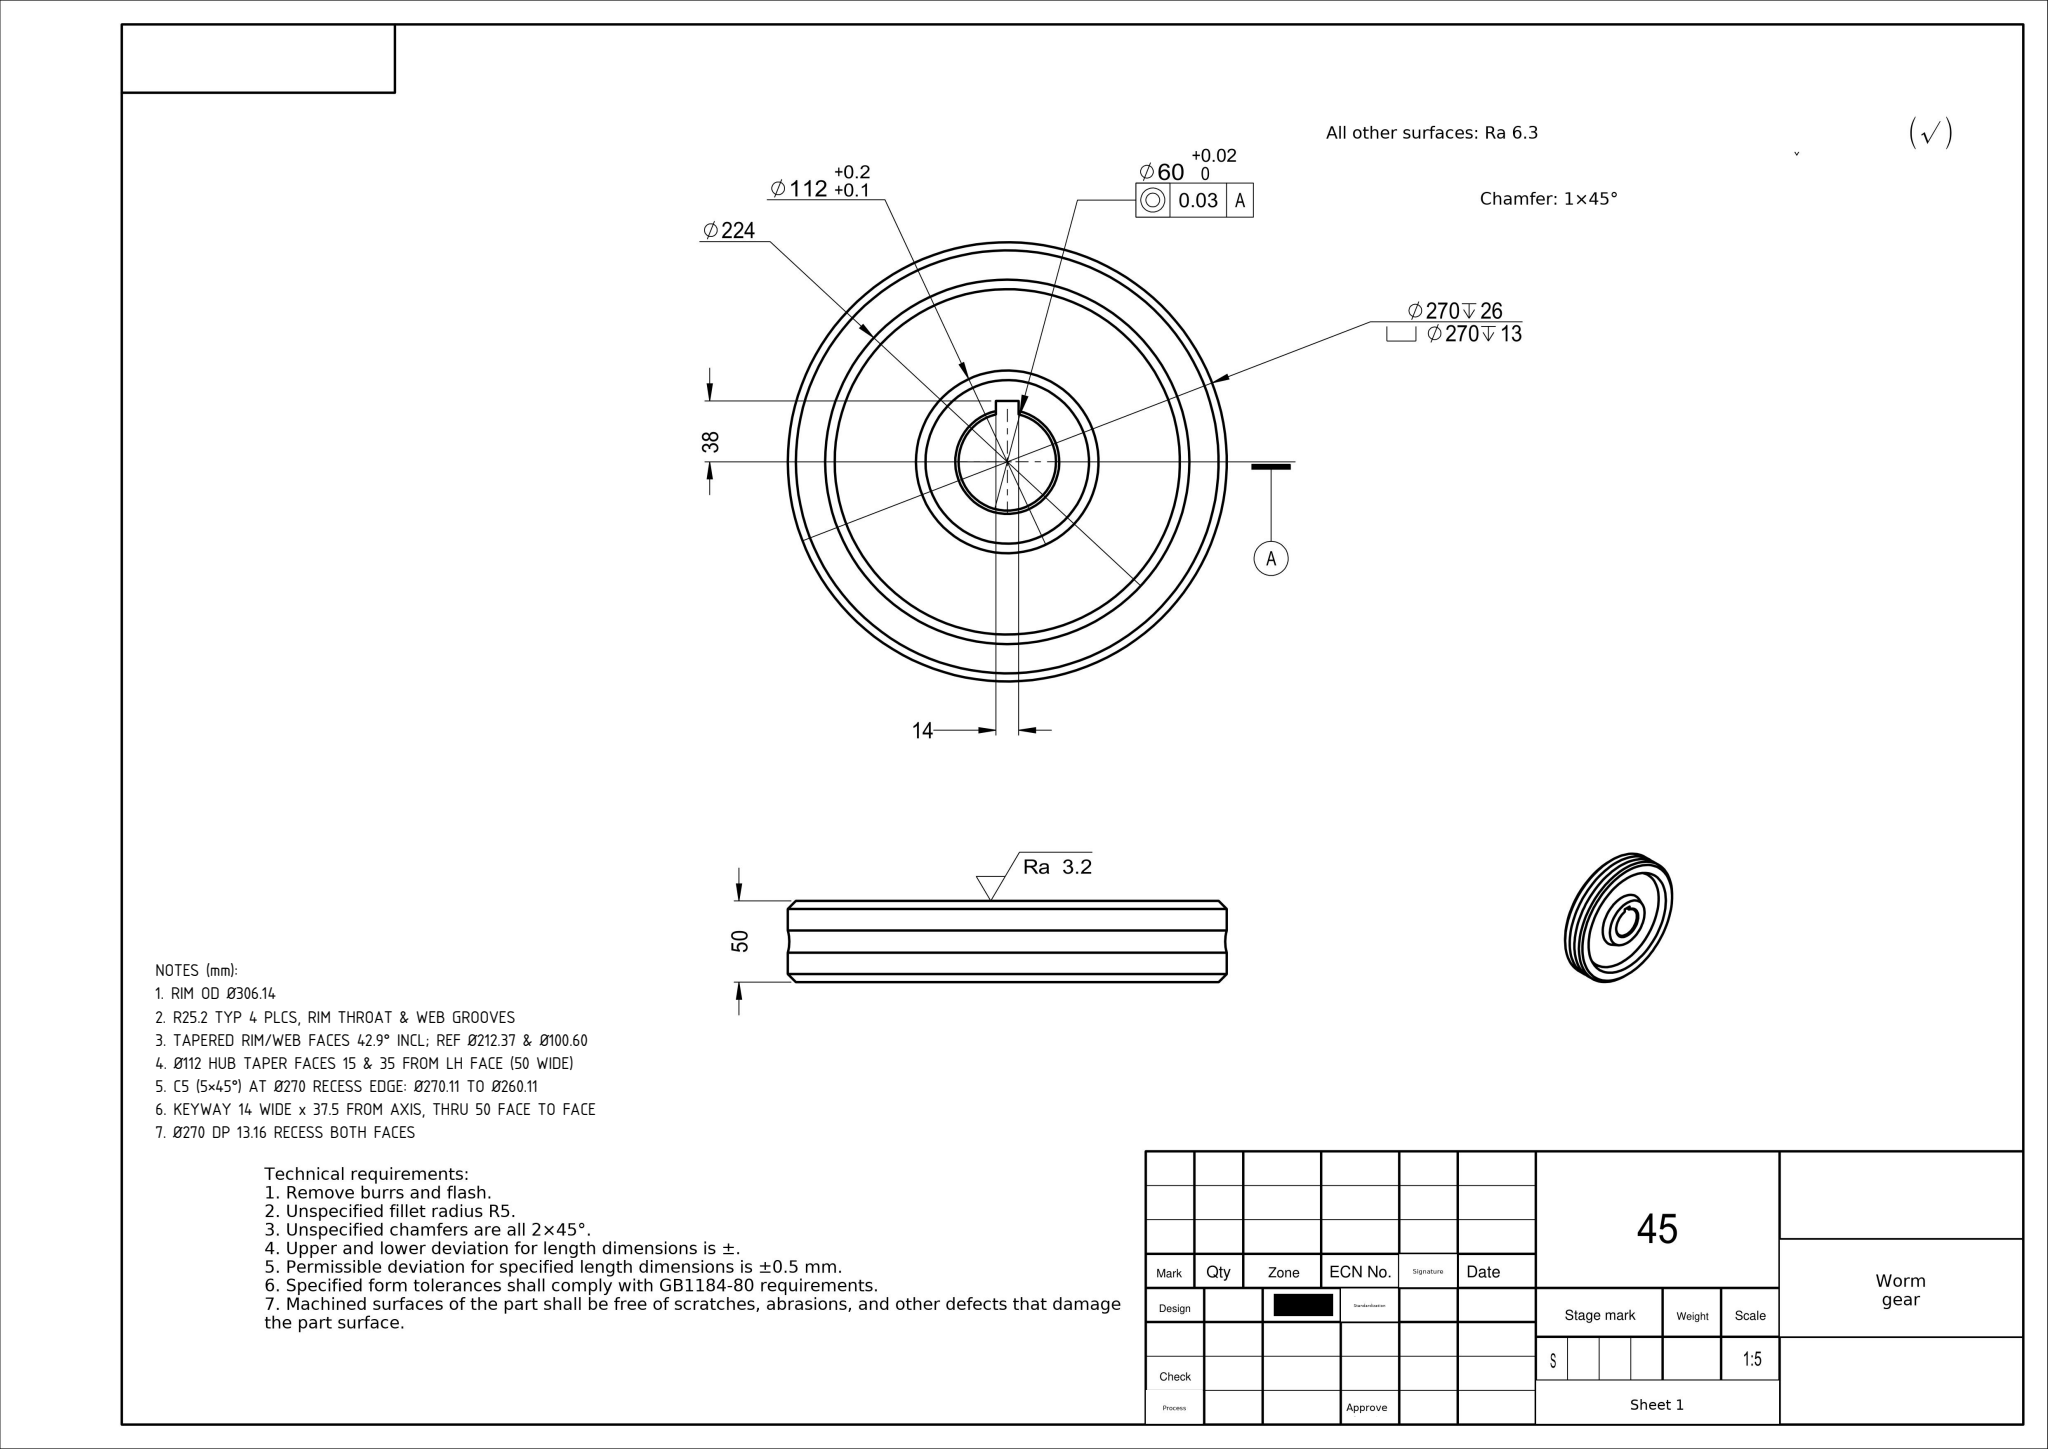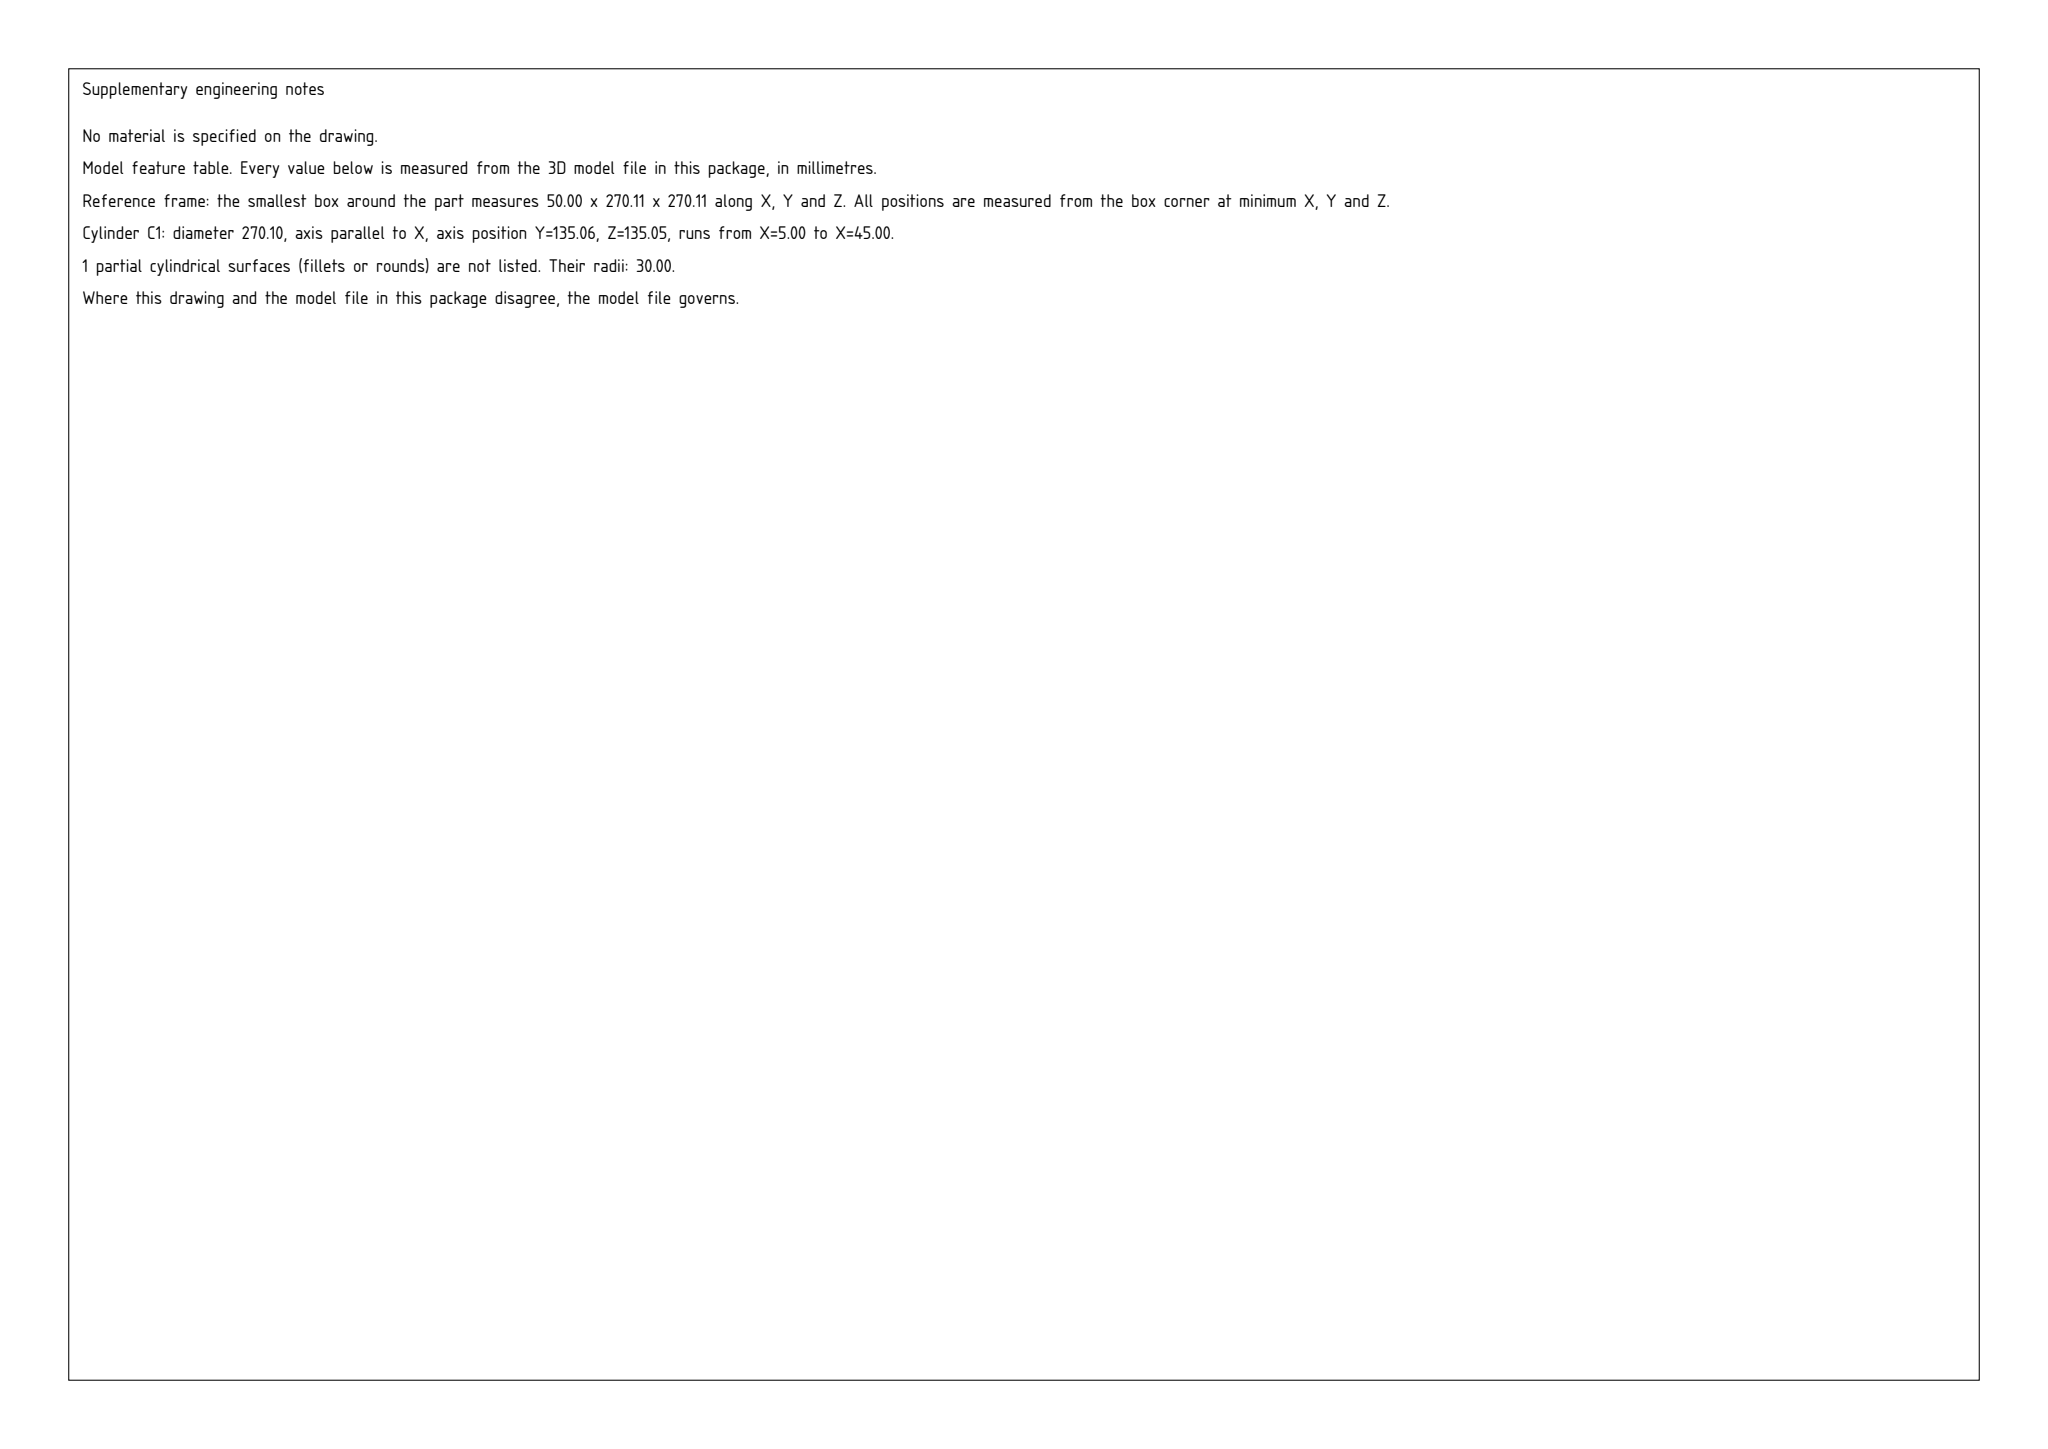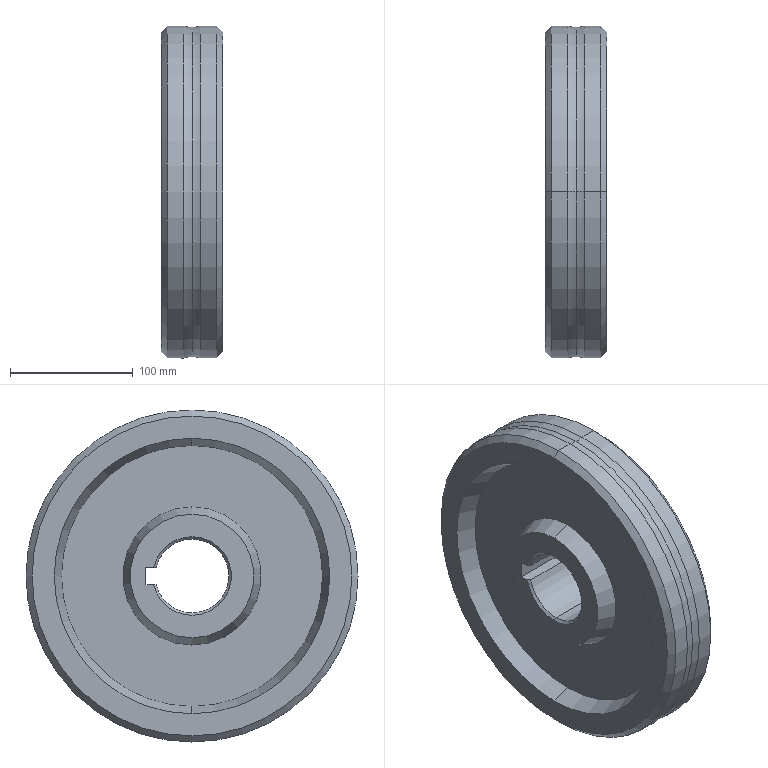Part | SolidWorks | mm | 1 solid | 38 faces | box 50 x 270.11 x 270.11 mm | volume 1834058 mm3 | cone 18 | plane 9 | cylinder 7 | torus 4 | commonest cylinder face diameters 270.108 x4 60 x3
Drawing notes:
RIM OD Ø306.14 | from the solid: bbox_xyz 306.138 across Y/Z = max outside dia
R25.2 TYP 4 PLCS, RIM THROAT & WEB GROOVES | from the solid: fillet_radii [25.2, count 4]
TAPERED RIM/WEB FACES 42.9° INCL; REF Ø212.37 & Ø100.60 | from the solid: cones [42.9,212.368,2] and [42.9,100.596,2]
Ø112 HUB TAPER FACES 15 & 35 FROM LH FACE (50 WIDE) | from the solid: axis_planes x=15, x=35; bbox x=50; cones [42.9,112.368]
C5 (5×45°) AT Ø270 RECESS EDGE: Ø270.11 TO Ø260.11 | from the solid: cones [90,270.108,2] & [90,260.108,2]; 5 radial drop
KEYWAY 14 WIDE x 37.5 FROM AXIS, THRU 50 FACE TO FACE | from the solid: z planes 146.07/160.07 (14 wide) abt axis 153.07; y 190.57-153.07=37.5; length 50
Ø270 DP 13.16 RECESS BOTH FACES | from the solid: cylinders [270.108,x,...,13.16,4]
build123d program:
from build123d import *

# Parameters (mm, degrees)
SKETCH3_W          = 14
SKETCH3_H          = 20.339
CUT_EXTRUDE1_DEPTH = 539.775


with BuildPart() as part:
    # Sketch2 → Revolve1 (revolve)
    with BuildSketch(Plane.XY, mode=Mode.PRIVATE) as revolve1_sk:
        with BuildLine():
            Line((2032.725, 352.117), (2032.725, 333.819))
            Line((2032.725, 333.819), (2047.725, 327.933))
            Line((2047.725, 327.933), (2047.725, 277.933))
            Line((2047.725, 277.933), (2032.725, 272.047))
            Line((2032.725, 272.047), (2032.725, 254.063))
            Line((2032.725, 254.063), (2037.725, 249.063))
            Line((2037.725, 249.063), (2050.889, 249.063))
            ThreePointArc((2050.889, 249.063), (2057.725, 250.008), (2064.562, 249.063))
            Line((2064.562, 249.063), (2077.725, 249.063))
            Line((2077.725, 249.063), (2082.725, 254.063))
            Line((2082.725, 254.063), (2082.725, 272.047))
            Line((2082.725, 272.047), (2067.725, 277.933))
            Line((2067.725, 277.933), (2067.725, 327.933))
            Line((2067.725, 327.933), (2082.725, 333.819))
            Line((2082.725, 333.819), (2082.725, 352.117))
            Line((2082.725, 352.117), (2080.725, 354.117))
            Line((2080.725, 354.117), (2034.725, 354.117))
            Line((2034.725, 354.117), (2032.725, 352.117))
        make_face()
    revolve(revolve1_sk.sketch.rotate(Axis((1797.706, 384.117, 0), (1, 0, 0)), 270), axis=Axis((1797.706, 384.117, 0), (1, 0, 0)))

    # Sketch3 → Cut-Extrude1 (cut, through all)
    with BuildSketch(Plane.ZY.offset(-2032.725)):
        with Locations((0, 411.448)):
            Rectangle(SKETCH3_W, SKETCH3_H)
    extrude(amount=-CUT_EXTRUDE1_DEPTH, mode=Mode.SUBTRACT)


solid = part.part